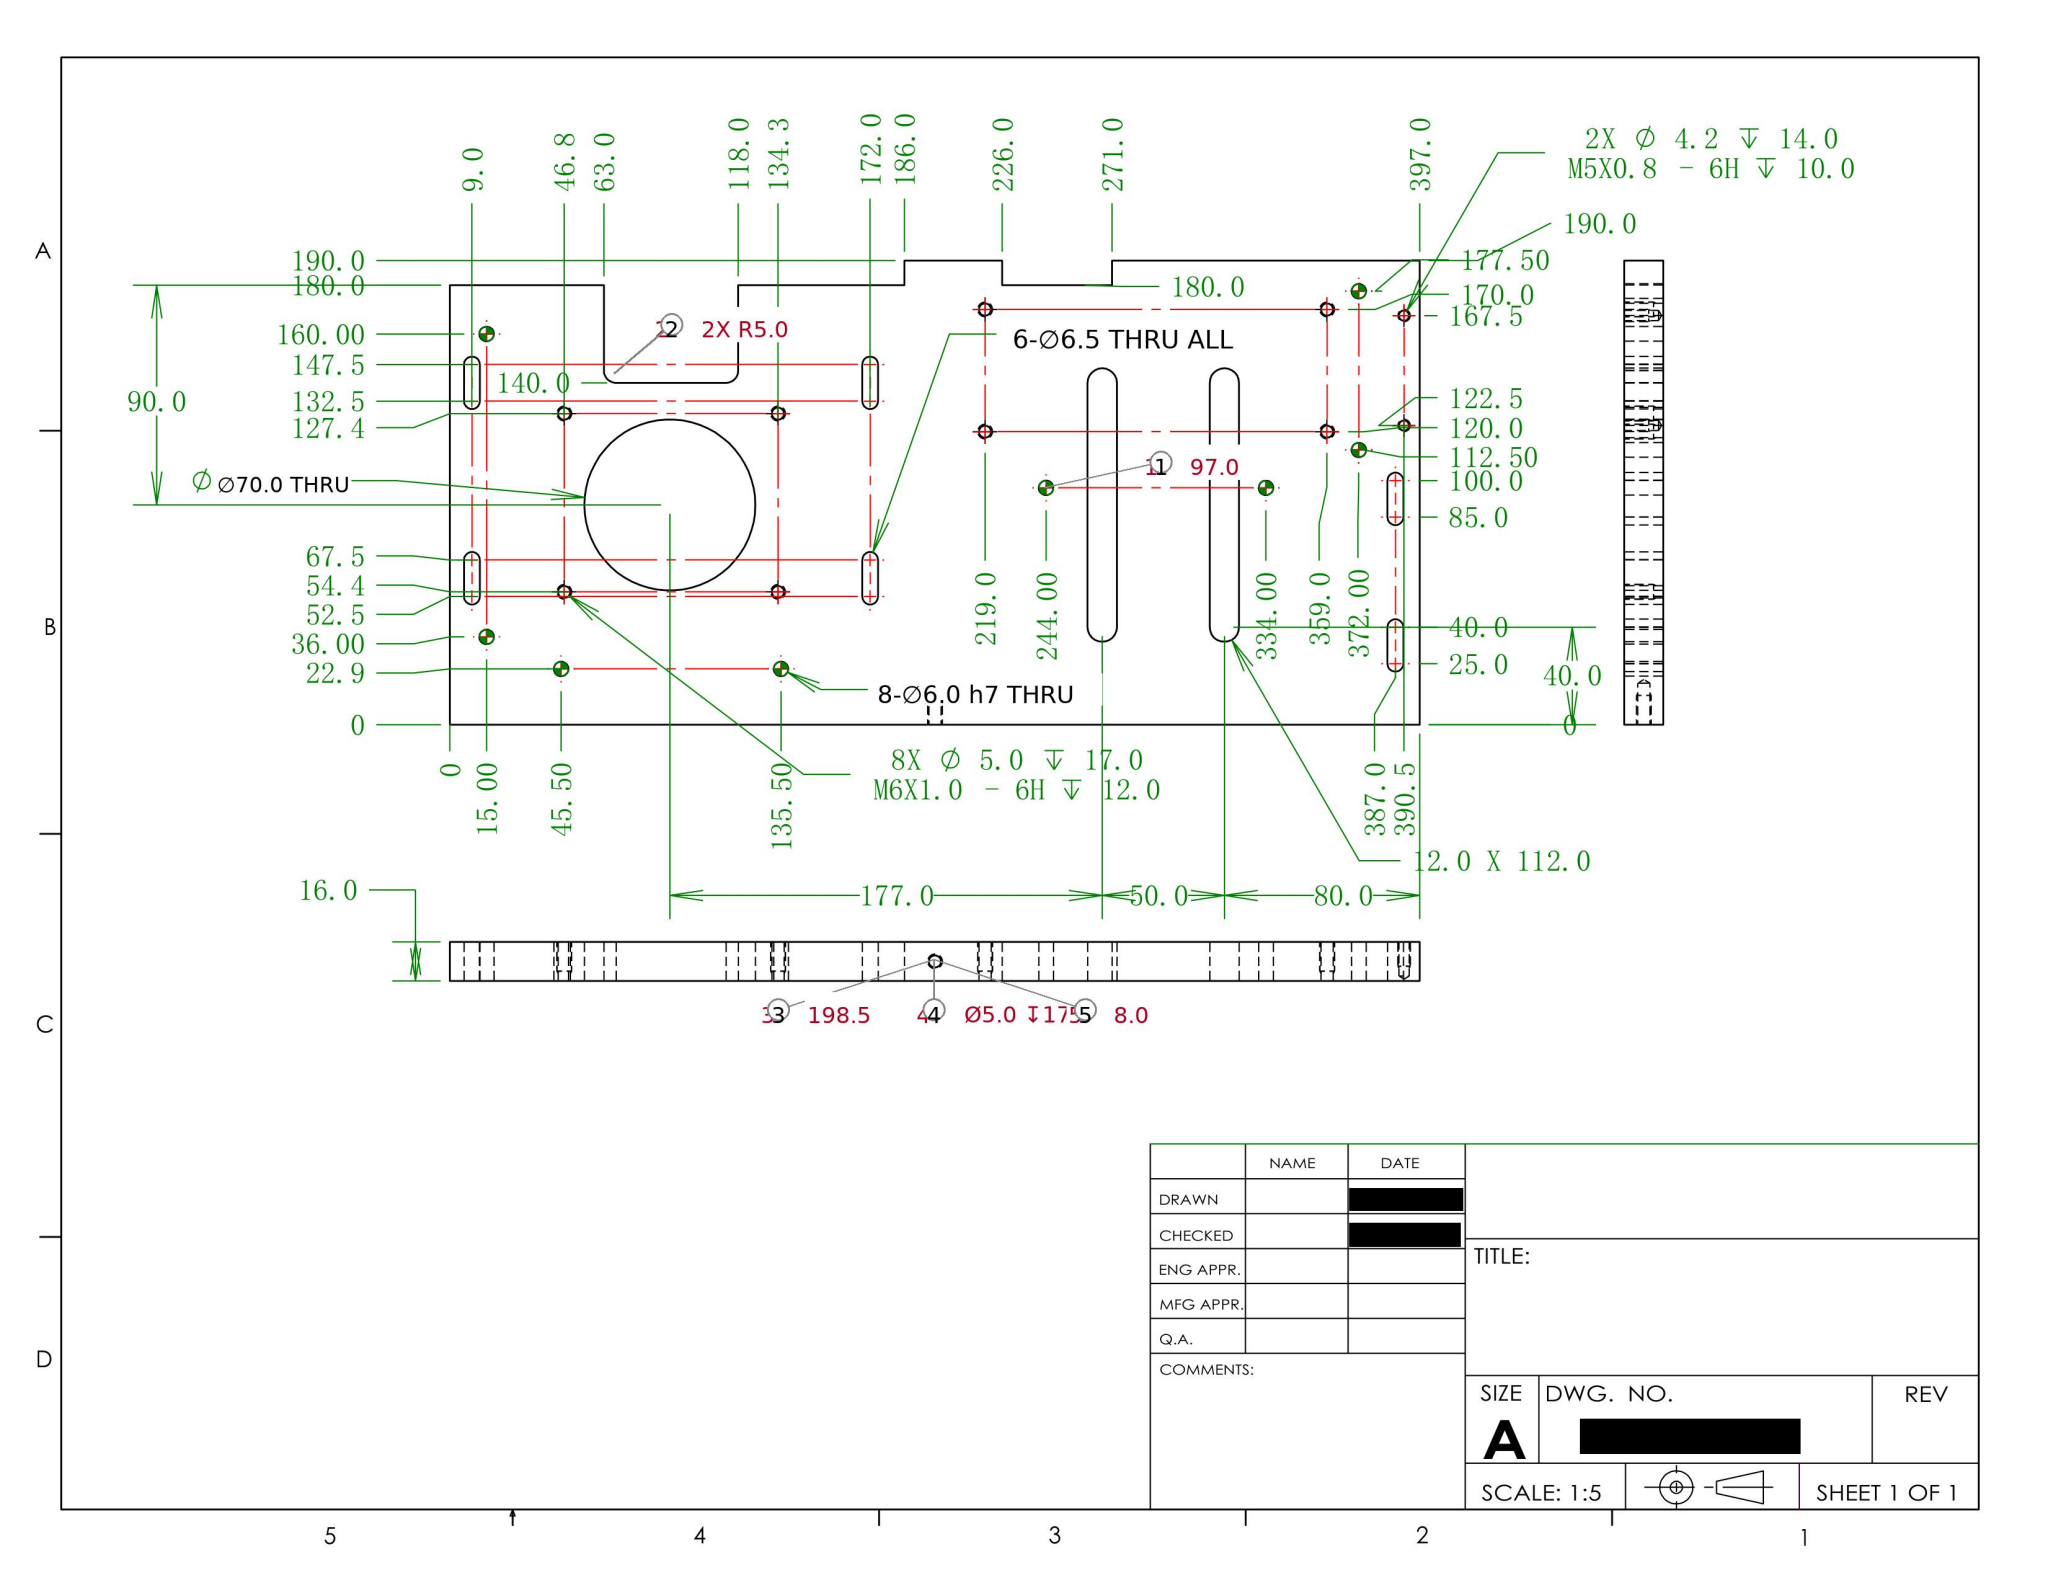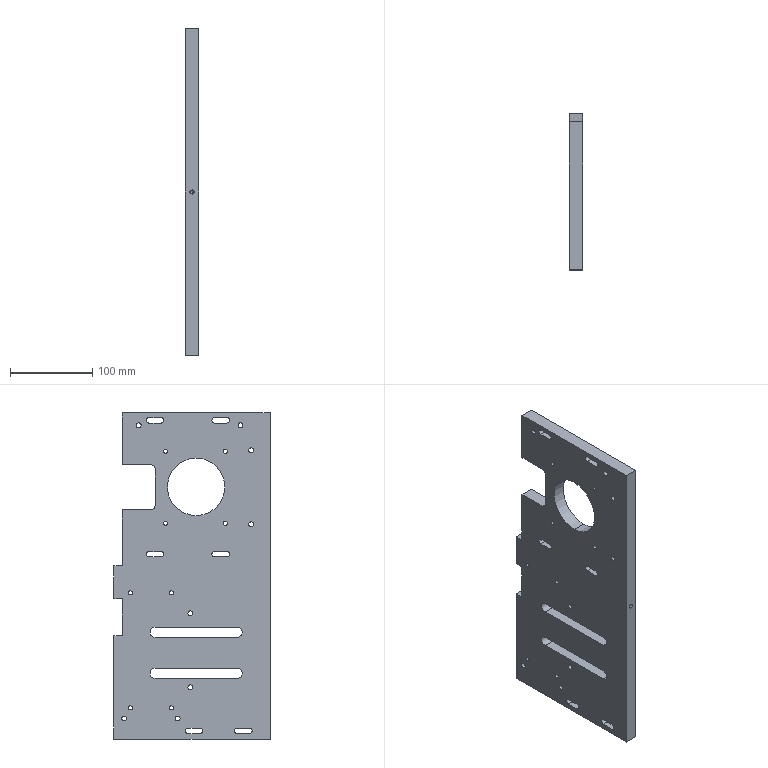Part | SolidWorks | mm | 1 solid | 96 faces | box 16 x 190 x 397 mm | volume 1011876 mm3 | cylinder 58 | plane 32 | cone 6 | commonest cylinder face diameters 5 x18 6 x16 6.5 x12 4.2 x4 12 x4 70 x2 10 x2
build123d program:
from build123d import *

# Parameters (mm, degrees)
SKETCH1_W                 = 400
SKETCH1_H                 = 230
EXTRUDE1_DEPTH            = 16
SKETCH2_W                 = 206.5
SKETCH2_H                 = 10
CUT_EXTRUDE1_DEPTH        = 462.688
SKETCH3_W                 = 55
SKETCH3_H                 = 40
SKETCH3_W_2               = 45
SKETCH3_H_2               = 10
CUT_EXTRUDE2_DEPTH        = 462.688
FILLET1_R                 = 5
M6X1_0_TAPPED_HOLE1_D     = 5
M6X1_0_TAPPED_HOLE1_DEPTH = 17
M6X1_0_TAPPED_HOLE1_TIP   = 1.502
SKETCH7_W                 = 16
SKETCH7_H                 = 220
CUT_EXTRUDE4_DEPTH        = 20.5
SKETCH8_W                 = 16
SKETCH8_H                 = 230
EXTRUDE2_DEPTH            = 2.5
SKETCH9_R                 = 3
CUT_EXTRUDE5_DEPTH        = 464.856
SKETCH10_W                = 16
SKETCH10_H                = 230
EXTRUDE3_DEPTH            = 15
M5X0_8_TAPPED_HOLE1_D     = 4.2
M5X0_8_TAPPED_HOLE1_DEPTH = 14
M5X0_8_TAPPED_HOLE1_TIP   = 1.262
SKETCH13_R                = 3
CUT_EXTRUDE6_DEPTH        = 477.93
M6X1_0_TAPPED_HOLE2_D     = 5
M6X1_0_TAPPED_HOLE2_DEPTH = 17
M6X1_0_TAPPED_HOLE2_TIP   = 1.502
SKETCH16_R                = 3
CUT_EXTRUDE7_DEPTH        = 477.93
SKETCH17_W                = 16
SKETCH17_H                = 397
CUT_EXTRUDE8_DEPTH        = 40
CUT_EXTRUDE9_DEPTH        = 477.93
M6X1_0_TAPPED_HOLE3_D     = 5
M6X1_0_TAPPED_HOLE3_DEPTH = 17
M6X1_0_TAPPED_HOLE3_TIP   = 1.502
SKETCH21_R                = 35
CUT_EXTRUDE10_DEPTH       = 477.93


with BuildPart() as part:
    # Sketch1 → Extrude1 (new body)
    with BuildSketch(Plane(origin=(0, 0, 0), x_dir=(0, 0, -1), z_dir=(1, 0, 0))):
        with Locations((200, 115)):
            Rectangle(SKETCH1_W, SKETCH1_H)
    extrude(amount=EXTRUDE1_DEPTH)

    # Sketch2 → Cut-Extrude1 (cut, through all)
    with BuildSketch(Plane(origin=(16, 0, 0), x_dir=(0, 0, -1), z_dir=(1, 0, 0))):
        with Locations((103.25, 225)):
            Rectangle(SKETCH2_W, SKETCH2_H)
    extrude(amount=-CUT_EXTRUDE1_DEPTH, mode=Mode.SUBTRACT)

    # Sketch3 → Cut-Extrude2 (cut, through all)
    with BuildSketch(Plane(origin=(16, 0, 0), x_dir=(0, 0, -1), z_dir=(1, 0, 0))):
        with Locations((111, 200)):
            Rectangle(SKETCH3_W, SKETCH3_H)
        with Locations((269, 225)):
            Rectangle(SKETCH3_W_2, SKETCH3_H_2)
    extrude(amount=-CUT_EXTRUDE2_DEPTH, mode=Mode.SUBTRACT)

    # Fillet1
    fillet1_edges = [part.edges().sort_by_distance(p)[0] for p in [
        (8, 180, -83.5),
        (8, 180, -138.5),
    ]]
    fillet(fillet1_edges, radius=FILLET1_R)

    # M6x1.0 Tapped Hole1
    with Locations(Plane(origin=(16, 0, 0), x_dir=(0, 0, -1), z_dir=(1, 0, 0))):
        with Locations((67.25, 167.4), (67.25, 94.4), (154.75, 167.4), (154.75, 94.4)):
            Hole(M6X1_0_TAPPED_HOLE1_D / 2, depth=M6X1_0_TAPPED_HOLE1_DEPTH)
            with Locations((0, 0, -(M6X1_0_TAPPED_HOLE1_DEPTH + M6X1_0_TAPPED_HOLE1_TIP / 2))):  # 118° drill point
                Cone(0, M6X1_0_TAPPED_HOLE1_D / 2, M6X1_0_TAPPED_HOLE1_TIP, mode=Mode.SUBTRACT)

    # Sketch7 → Cut-Extrude4 (cut)
    with BuildSketch(Plane.XY):
        with Locations((8, 110)):
            Rectangle(SKETCH7_W, SKETCH7_H)
    extrude(amount=-CUT_EXTRUDE4_DEPTH, mode=Mode.SUBTRACT)

    # Sketch8 → Extrude2 (add)
    with BuildSketch(Plane(origin=(0, 0, -400), x_dir=(-1, 0, 0), z_dir=(0, 0, -1))):
        with Locations((-8, 115)):
            Rectangle(SKETCH8_W, SKETCH8_H)
    extrude(amount=EXTRUDE2_DEPTH)

    # Sketch9 → Cut-Extrude5 (cut, through all)
    with BuildSketch(Plane(origin=(16, 0, 0), x_dir=(0, 0, -1), z_dir=(1, 0, 0))):
        with Locations((66, 62.9)):
            Circle(SKETCH9_R)
        with Locations((156, 62.9)):
            Circle(SKETCH9_R)
        with Locations((264.5, 137)):
            Circle(SKETCH9_R)
        with Locations((354.5, 137)):
            Circle(SKETCH9_R)
    extrude(amount=-CUT_EXTRUDE5_DEPTH, mode=Mode.SUBTRACT)

    # Sketch10 → Extrude3 (add)
    with BuildSketch(Plane(origin=(0, 0, -402.5), x_dir=(-1, 0, 0), z_dir=(0, 0, -1))):
        with Locations((-8, 115)):
            Rectangle(SKETCH10_W, SKETCH10_H)
    extrude(amount=EXTRUDE3_DEPTH)

    # M5x0.8 Tapped Hole1
    with Locations(Plane(origin=(16, 0, 0), x_dir=(0, 0, -1), z_dir=(1, 0, 0))):
        with Locations((411, 207.5), (411, 162.5)):
            Hole(M5X0_8_TAPPED_HOLE1_D / 2, depth=M5X0_8_TAPPED_HOLE1_DEPTH)
            with Locations((0, 0, -(M5X0_8_TAPPED_HOLE1_DEPTH + M5X0_8_TAPPED_HOLE1_TIP / 2))):  # 118° drill point
                Cone(0, M5X0_8_TAPPED_HOLE1_D / 2, M5X0_8_TAPPED_HOLE1_TIP, mode=Mode.SUBTRACT)

    # Sketch13 → Cut-Extrude6 (cut, through all)
    with BuildSketch(Plane(origin=(16, 0, 0), x_dir=(0, 0, -1), z_dir=(1, 0, 0))):
        with Locations((392.5, 217.5)):
            Circle(SKETCH13_R)
        with Locations((392.5, 152.5)):
            Circle(SKETCH13_R)
    extrude(amount=-CUT_EXTRUDE6_DEPTH, mode=Mode.SUBTRACT)

    # M6x1.0 Tapped Hole2
    with Locations(Plane(origin=(16, 0, 0), x_dir=(0, 0, -1), z_dir=(1, 0, 0))):
        with Locations((239.5, 210), (239.5, 160), (379.5, 160), (379.5, 210)):
            Hole(M6X1_0_TAPPED_HOLE2_D / 2, depth=M6X1_0_TAPPED_HOLE2_DEPTH)
            with Locations((0, 0, -(M6X1_0_TAPPED_HOLE2_DEPTH + M6X1_0_TAPPED_HOLE2_TIP / 2))):  # 118° drill point
                Cone(0, M6X1_0_TAPPED_HOLE2_D / 2, M6X1_0_TAPPED_HOLE2_TIP, mode=Mode.SUBTRACT)

    # Sketch16 → Cut-Extrude7 (cut, through all)
    with BuildSketch(Plane(origin=(16, 0, 0), x_dir=(0, 0, -1), z_dir=(1, 0, 0))):
        with Locations((35.5, 200)):
            Circle(SKETCH16_R)
        with Locations((35.5, 76)):
            Circle(SKETCH16_R)
    extrude(amount=-CUT_EXTRUDE7_DEPTH, mode=Mode.SUBTRACT)

    # Sketch17 → Cut-Extrude8 (cut)
    with BuildSketch(Plane.XZ):
        with Locations((8, -219)):
            Rectangle(SKETCH17_W, SKETCH17_H)
    extrude(amount=-CUT_EXTRUDE8_DEPTH, mode=Mode.SUBTRACT)

    # Sketch18 → Cut-Extrude9 (cut, through all)
    with BuildSketch(Plane(origin=(16, 0, 0), x_dir=(0, 0, -1), z_dir=(1, 0, 0))):
        with BuildLine():
            Line((32.75, 187.5), (32.75, 172.5))
            ThreePointArc((32.75, 172.5), (29.5, 169.25), (26.25, 172.5))
            Line((26.25, 172.5), (26.25, 187.5))
            ThreePointArc((26.25, 187.5), (29.5, 190.75), (32.75, 187.5))
        make_face()
        with BuildLine():
            Line((32.75, 107.5), (32.75, 92.5))
            ThreePointArc((32.75, 92.5), (29.5, 89.25), (26.25, 92.5))
            Line((26.25, 92.5), (26.25, 107.5))
            ThreePointArc((26.25, 107.5), (29.5, 110.75), (32.75, 107.5))
        make_face()
        with BuildLine():
            Line((195.75, 187.5), (195.75, 172.5))
            ThreePointArc((195.75, 172.5), (192.5, 169.25), (189.25, 172.5))
            Line((189.25, 172.5), (189.25, 187.5))
            ThreePointArc((189.25, 187.5), (192.5, 190.75), (195.75, 187.5))
        make_face()
        with BuildLine():
            Line((195.75, 107.5), (195.75, 92.5))
            ThreePointArc((195.75, 92.5), (192.5, 89.25), (189.25, 92.5))
            Line((189.25, 92.5), (189.25, 107.5))
            ThreePointArc((189.25, 107.5), (192.5, 110.75), (195.75, 107.5))
        make_face()
        with BuildLine():
            Line((410.75, 140), (410.75, 125))
            ThreePointArc((410.75, 125), (407.5, 121.75), (404.25, 125))
            Line((404.25, 125), (404.25, 140))
            ThreePointArc((404.25, 140), (407.5, 143.25), (410.75, 140))
        make_face()
        with BuildLine():
            Line((410.75, 80), (410.75, 65))
            ThreePointArc((410.75, 65), (407.5, 61.75), (404.25, 65))
            Line((404.25, 65), (404.25, 80))
            ThreePointArc((404.25, 80), (407.5, 83.25), (410.75, 80))
        make_face()
    extrude(amount=-CUT_EXTRUDE9_DEPTH, mode=Mode.SUBTRACT)

    # M6x1.0 Tapped Hole3
    with Locations(Plane.XZ.offset(-40)):
        with Locations((8, -219)):
            Hole(M6X1_0_TAPPED_HOLE3_D / 2, depth=M6X1_0_TAPPED_HOLE3_DEPTH)
            with Locations((0, 0, -(M6X1_0_TAPPED_HOLE3_DEPTH + M6X1_0_TAPPED_HOLE3_TIP / 2))):  # 118° drill point
                Cone(0, M6X1_0_TAPPED_HOLE3_D / 2, M6X1_0_TAPPED_HOLE3_TIP, mode=Mode.SUBTRACT)

    # Sketch21 → Cut-Extrude10 (cut, through all)
    with BuildSketch(Plane(origin=(16, 0, 0), x_dir=(0, 0, -1), z_dir=(1, 0, 0))):
        with Locations((110.5, 130)):
            Circle(SKETCH21_R)
        with BuildLine():
            Line((293.5, 180), (293.5, 80))
            ThreePointArc((293.5, 80), (287.5, 74), (281.5, 80))
            Line((281.5, 80), (281.5, 180))
            ThreePointArc((281.5, 180), (287.5, 186), (293.5, 180))
        make_face()
        with BuildLine():
            Line((343.5, 180), (343.5, 80))
            ThreePointArc((343.5, 80), (337.5, 74), (331.5, 80))
            Line((331.5, 80), (331.5, 180))
            ThreePointArc((331.5, 180), (337.5, 186), (343.5, 180))
        make_face()
    extrude(amount=-CUT_EXTRUDE10_DEPTH, mode=Mode.SUBTRACT)


solid = part.part